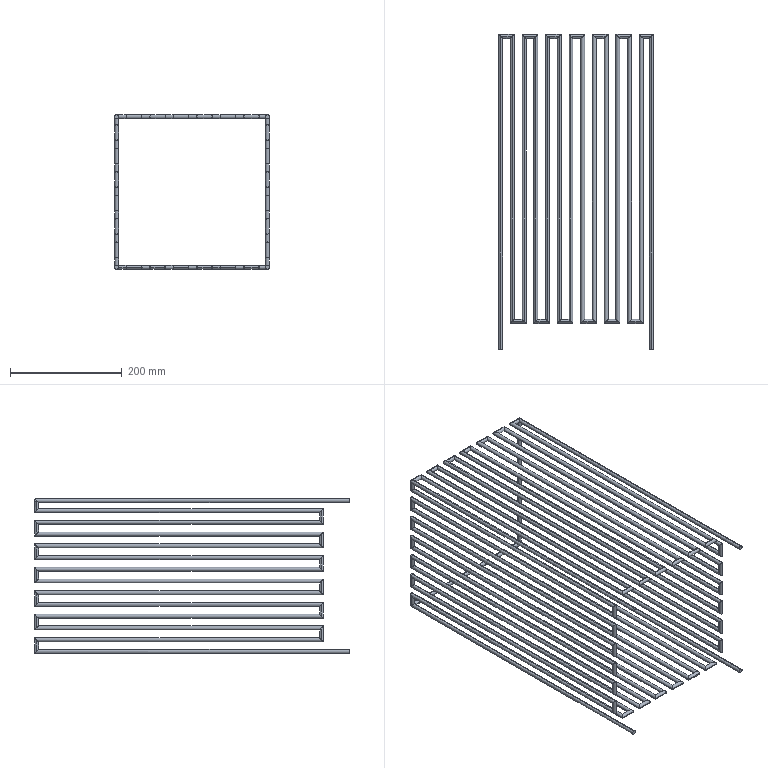Component | SolidWorks | InsectTrapLamp-1_ElectricNet-1 | 1 solid | 214 faces | box 277 x 563.5 x 277 mm | volume 1069412 mm3 | cylinder 210 | plane 4 | commonest cylinder face diameters 7 x210
build123d program:
from build123d import *

# Parameters (mm, degrees)
SWEEP4_PROFILE_R = 3.5
SWEEP5_PROFILE_R = 3.5
SWEEP6_PROFILE_R = 3.5
SWEEP7_PROFILE_R = 3.5


with BuildPart() as part:
    # Sweep4: sweep along a curve in space
    with BuildLine() as sweep4_path:
        Line((-135, 0, 135), (-135, 560, 135))
        Line((-135, 560, 135), (-114, 560, 135))
        Line((-114, 560, 135), (-114, 50, 135))
        Line((-114, 50, 135), (-93, 50, 135))
        Line((-93, 50, 135), (-93, 560, 135))
        Line((-93, 560, 135), (-72, 560, 135))
        Line((-72, 560, 135), (-72, 50, 135))
        Line((-72, 50, 135), (-51, 50, 135))
        Line((-51, 50, 135), (-51, 560, 135))
        Line((-51, 560, 135), (-30, 560, 135))
        Line((-30, 560, 135), (-30, 50, 135))
        Line((-30, 50, 135), (-9, 50, 135))
        Line((-9, 50, 135), (-9, 560, 135))
        Line((-9, 560, 135), (12, 560, 135))
        Line((12, 560, 135), (12, 50, 135))
        Line((12, 50, 135), (33, 50, 135))
        Line((33, 50, 135), (33, 560, 135))
        Line((33, 560, 135), (54, 560, 135))
        Line((54, 560, 135), (54, 50, 135))
        Line((54, 50, 135), (75, 50, 135))
        Line((75, 50, 135), (75, 560, 135))
        Line((75, 560, 135), (96, 560, 135))
        Line((96, 560, 135), (96, 50, 135))
        Line((96, 50, 135), (117, 50, 135))
        Line((117, 50, 135), (117, 560, 135))
        Line((117, 560, 135), (135, 560, 135))
        Line((135, 0, 135), (135, 560, 135))
    # Sweep4 profile (on start of the path) → Sweep4 (sweep)
    with BuildSketch(Plane(origin=(-135, 0, 135), x_dir=(0, 0, 1), z_dir=(0, 1, 0))):
        Circle(SWEEP4_PROFILE_R)
    sweep(path=sweep4_path.line, transition=Transition.RIGHT)

    # Sweep5: sweep along a curve in space
    with BuildLine() as sweep5_path:
        Line((-135, 560, 117), (-135, 560, 135))
        Line((-135, 50, 117), (-135, 560, 117))
        Line((-135, 50, 96), (-135, 50, 117))
        Line((-135, 560, 96), (-135, 50, 96))
        Line((-135, 560, 75), (-135, 560, 96))
        Line((-135, 50, 75), (-135, 560, 75))
        Line((-135, 50, 54), (-135, 50, 75))
        Line((-135, 560, 54), (-135, 50, 54))
        Line((-135, 560, 33), (-135, 560, 54))
        Line((-135, 50, 33), (-135, 560, 33))
        Line((-135, 50, 12), (-135, 50, 33))
        Line((-135, 560, 12), (-135, 50, 12))
        Line((-135, 560, -9), (-135, 560, 12))
        Line((-135, 50, -9), (-135, 560, -9))
        Line((-135, 50, -30), (-135, 50, -9))
        Line((-135, 560, -30), (-135, 50, -30))
        Line((-135, 560, -51), (-135, 560, -30))
        Line((-135, 50, -51), (-135, 560, -51))
        Line((-135, 50, -72), (-135, 50, -51))
        Line((-135, 560, -72), (-135, 50, -72))
        Line((-135, 560, -93), (-135, 560, -72))
        Line((-135, 50, -93), (-135, 560, -93))
        Line((-135, 50, -114), (-135, 50, -93))
        Line((-135, 560, -114), (-135, 50, -114))
        Line((-135, 560, -135), (-135, 560, -114))
        Line((-135, 0, -135), (-135, 560, -135))
    # Sweep5 profile (on start of the path) → Sweep5 (sweep)
    with BuildSketch(Plane(origin=(-135, 0, -135), x_dir=(0, 0, 1), z_dir=(0, 1, 0))):
        Circle(SWEEP5_PROFILE_R)
    sweep(path=sweep5_path.line, transition=Transition.RIGHT)

    # Sweep6: sweep along a path in Sketch3
    with BuildLine(Plane(origin=(135, 0, 0), x_dir=(0, 0, -1), z_dir=(1, 0, 0))) as sweep6_path:
        Line((-135, 560), (-117, 560))
        Line((-117, 560), (-117, 50))
        Line((-117, 50), (-96, 50))
        Line((-96, 50), (-96, 560))
        Line((-96, 560), (-75, 560))
        Line((-75, 560), (-75, 50))
        Line((-75, 50), (-54, 50))
        Line((-54, 50), (-54, 560))
        Line((-54, 560), (-33, 560))
        Line((-33, 560), (-33, 50))
        Line((-33, 50), (-12, 50))
        Line((-12, 50), (-12, 560))
        Line((-12, 560), (9, 560))
        Line((9, 560), (9, 50))
        Line((9, 50), (30, 50))
        Line((30, 50), (30, 560))
        Line((30, 560), (51, 560))
        Line((51, 560), (51, 50))
        Line((51, 50), (72, 50))
        Line((72, 50), (72, 560))
        Line((72, 560), (93, 560))
        Line((93, 560), (93, 50))
        Line((93, 50), (114, 50))
        Line((114, 50), (114, 560))
        Line((114, 560), (135, 560))
        Line((135, 560), (135, 0))
    # Sweep6 profile (on start of the path) → Sweep6 (sweep)
    with BuildSketch(Plane(origin=(135, 560, 135), x_dir=(-1, 0, 0), z_dir=(0, 0, -1))):
        Circle(SWEEP6_PROFILE_R)
    sweep(path=sweep6_path.line, transition=Transition.RIGHT)

    # Sweep7: sweep along a path in Sketch4
    with BuildLine(Plane.XY.offset(-135)) as sweep7_path:
        Line((-135, 560), (-114, 560))
        Line((-114, 560), (-114, 50))
        Line((-114, 50), (-93, 50))
        Line((-93, 50), (-93, 560))
        Line((-93, 560), (-72, 560))
        Line((-72, 560), (-72, 50))
        Line((-72, 50), (-51, 50))
        Line((-51, 50), (-51, 560))
        Line((-51, 560), (-30, 560))
        Line((-30, 560), (-30, 50))
        Line((-30, 50), (-9, 50))
        Line((-9, 50), (-9, 560))
        Line((-9, 560), (12, 560))
        Line((12, 560), (12, 50))
        Line((12, 50), (33, 50))
        Line((33, 50), (33, 560))
        Line((33, 560), (54, 560))
        Line((54, 560), (54, 50))
        Line((54, 50), (75, 50))
        Line((75, 50), (75, 560))
        Line((75, 560), (96, 560))
        Line((96, 560), (96, 50))
        Line((96, 50), (117, 50))
        Line((117, 50), (117, 560))
        Line((117, 560), (135, 560))
    # Sweep7 profile (on start of the path) → Sweep7 (sweep)
    with BuildSketch(Plane(origin=(-135, 560, -135), x_dir=(0, 1, 0), z_dir=(1, 0, 0))):
        Circle(SWEEP7_PROFILE_R)
    sweep(path=sweep7_path.line, transition=Transition.RIGHT)


solid = part.part

# Placed as in the assembly
solid = solid.moved(Location((0, 880.001, 0), (0, 0, 0)))